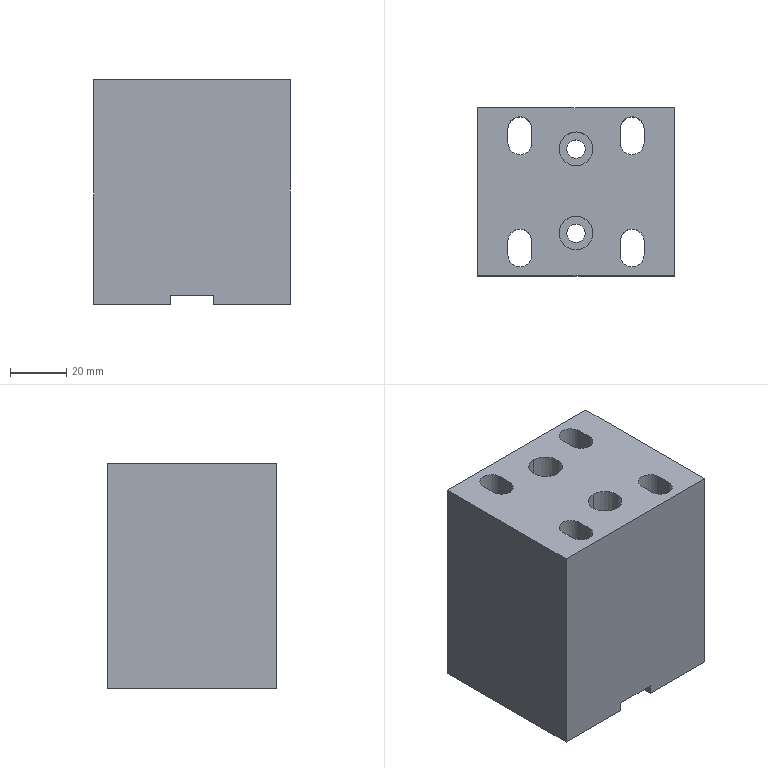Component | SolidWorks | 2SZT-0-004-1 | 1 solid | 40 faces | box 70 x 60 x 80 mm | volume 286633 mm3 | cylinder 20 | plane 20 | commonest cylinder face diameters 8.5 x12 12 x4 6.5 x4
build123d program:
from build123d import *

# Parameters (mm, degrees)
SKETCH1_W                                            = 70
SKETCH1_H                                            = 90
BOSS_EXTRUDE1_DEPTH                                  = 80
SKETCH2_W                                            = 64
SKETCH2_H                                            = 79.442
CUT_EXTRUDE1_DEPTH                                   = 1.5
SKETCH8_W                                            = 15
SKETCH8_H                                            = 167.061
CUT_EXTRUDE2_DEPTH                                   = 3.25
HOLE_SIZE_ACCORDING_TO_THE_TYPE_OF_HEXAG_D           = 6.5
HOLE_SIZE_ACCORDING_TO_THE_TYPE_OF_HEXAG_CBORE_D     = 12
HOLE_SIZE_ACCORDING_TO_THE_TYPE_OF_HEXAG_CBORE_DEPTH = 60
F_6_0_6_DIAMETER_HOLE1_D                             = 6.01
F_6_0_6_DIAMETER_HOLE1_DEPTH                         = 89.33
F_6_0_6_DIAMETER_HOLE1_TIP                           = 1.806
M4_TAPPED_HOLE1_D                                    = 3.3
M4_TAPPED_HOLE1_DEPTH                                = 10.1
M4_TAPPED_HOLE1_TIP                                  = 0.9914
CUT_EXTRUDE4_DEPTH                                   = 99.234
SKETCH25_W                                           = 188.53
SKETCH25_H                                           = 35.448
CUT_EXTRUDE5_DEPTH                                   = 30
SKETCH26_W                                           = 83.621
SKETCH26_H                                           = 63.514
CUT_EXTRUDE6_DEPTH                                   = 100


with BuildPart() as part:
    # Sketch1 → Boss-Extrude1 (new body)
    with BuildSketch(Plane(origin=(0, 0, 0), x_dir=(1, 0, 0), z_dir=(0, 1, 0))):
        Rectangle(SKETCH1_W, SKETCH1_H)
    extrude(amount=BOSS_EXTRUDE1_DEPTH)

    # Sketch2 → Cut-Extrude1 (cut)
    with BuildSketch(Plane(origin=(0, 0, -45), x_dir=(-1, 0, 0), z_dir=(0, 0, -1))):
        with Locations((0, 66.041)):
            Rectangle(SKETCH2_W, SKETCH2_H)
    extrude(amount=-CUT_EXTRUDE1_DEPTH, mode=Mode.SUBTRACT)

    # Sketch8 → Cut-Extrude2 (cut)
    with BuildSketch(Plane(origin=(0, 80, 0), x_dir=(1, 0, 0), z_dir=(0, 1, 0))):
        Rectangle(SKETCH8_W, SKETCH8_H)
    extrude(amount=-CUT_EXTRUDE2_DEPTH, mode=Mode.SUBTRACT)

    # Hole Size according to the type of hexag (through all)
    with Locations(Plane.XZ):
        with Locations((0, 29.657), (0, -0.3432)):
            CounterBoreHole(HOLE_SIZE_ACCORDING_TO_THE_TYPE_OF_HEXAG_D / 2, HOLE_SIZE_ACCORDING_TO_THE_TYPE_OF_HEXAG_CBORE_D / 2, HOLE_SIZE_ACCORDING_TO_THE_TYPE_OF_HEXAG_CBORE_DEPTH)

    # 6.0 _6_ Diameter Hole1
    with Locations(Plane(origin=(0, 80, 0), x_dir=(-1, 0, 0), z_dir=(0, 1, 0))):
        with Locations((20, 35), (20, -5), (-20, -5), (-20, 35)):
            Hole(F_6_0_6_DIAMETER_HOLE1_D / 2, depth=F_6_0_6_DIAMETER_HOLE1_DEPTH)
            with Locations((0, 0, -(F_6_0_6_DIAMETER_HOLE1_DEPTH + F_6_0_6_DIAMETER_HOLE1_TIP / 2))):  # 118° drill point
                Cone(0, F_6_0_6_DIAMETER_HOLE1_D / 2, F_6_0_6_DIAMETER_HOLE1_TIP, mode=Mode.SUBTRACT)

    # M4 Tapped Hole1
    with Locations(Plane(origin=(0, 0, -43.5), x_dir=(-1, 0, 0), z_dir=(0, 0, -1))):
        with Locations((-12, 40.32), (12, 40.32), (12, 64.32), (-12, 64.32)):
            Hole(M4_TAPPED_HOLE1_D / 2, depth=M4_TAPPED_HOLE1_DEPTH)
            with Locations((0, 0, -(M4_TAPPED_HOLE1_DEPTH + M4_TAPPED_HOLE1_TIP / 2))):  # 118° drill point
                Cone(0, M4_TAPPED_HOLE1_D / 2, M4_TAPPED_HOLE1_TIP, mode=Mode.SUBTRACT)

    # Sketch24 → Cut-Extrude4 (cut, through all)
    with BuildSketch(Plane(origin=(0, 80, 0), x_dir=(1, 0, 0), z_dir=(0, 1, 0))):
        with BuildLine():
            Line((-24.25, 2.5), (-24.25, 7.5))
            ThreePointArc((-24.25, 7.5), (-20, 11.75), (-15.75, 7.5))
            Line((-15.75, 7.5), (-15.75, 2.5))
            ThreePointArc((-15.75, 2.5), (-20, -1.75), (-24.25, 2.5))
        make_face()
        with BuildLine():
            Line((15.75, 2.5), (15.75, 7.5))
            ThreePointArc((15.75, 7.5), (20, 11.75), (24.25, 7.5))
            Line((24.25, 7.5), (24.25, 2.5))
            ThreePointArc((24.25, 2.5), (20, -1.75), (15.75, 2.5))
        make_face()
        with BuildLine():
            Line((15.75, -37.5), (15.75, -32.5))
            ThreePointArc((15.75, -32.5), (20, -28.25), (24.25, -32.5))
            Line((24.25, -32.5), (24.25, -37.5))
            ThreePointArc((24.25, -37.5), (20, -41.75), (15.75, -37.5))
        make_face()
        with BuildLine():
            Line((-24.25, -37.5), (-24.25, -32.5))
            ThreePointArc((-24.25, -32.5), (-20, -28.25), (-15.75, -32.5))
            Line((-15.75, -32.5), (-15.75, -37.5))
            ThreePointArc((-15.75, -37.5), (-20, -41.75), (-24.25, -37.5))
        make_face()
    extrude(amount=-CUT_EXTRUDE4_DEPTH, mode=Mode.SUBTRACT)

    # Sketch25 → Cut-Extrude5 (cut)
    with BuildSketch(Plane(origin=(0, 0, -45), x_dir=(-1, 0, 0), z_dir=(0, 0, -1))):
        with Locations((-5.629, 85.724)):
            Rectangle(SKETCH25_W, SKETCH25_H)
    extrude(amount=-CUT_EXTRUDE5_DEPTH, mode=Mode.SUBTRACT)

    # Sketch26 → Cut-Extrude6 (cut)
    with BuildSketch(Plane(origin=(0, 68, 0), x_dir=(1, 0, 0), z_dir=(0, 1, 0))):
        with Locations((6.81, 46.757)):
            Rectangle(SKETCH26_W, SKETCH26_H)
    extrude(amount=-CUT_EXTRUDE6_DEPTH, mode=Mode.SUBTRACT)


solid = part.part

# Placed as in the assembly
solid = solid.moved(Location((955.268, 332.75, -175.946), (90, 0, -180)))